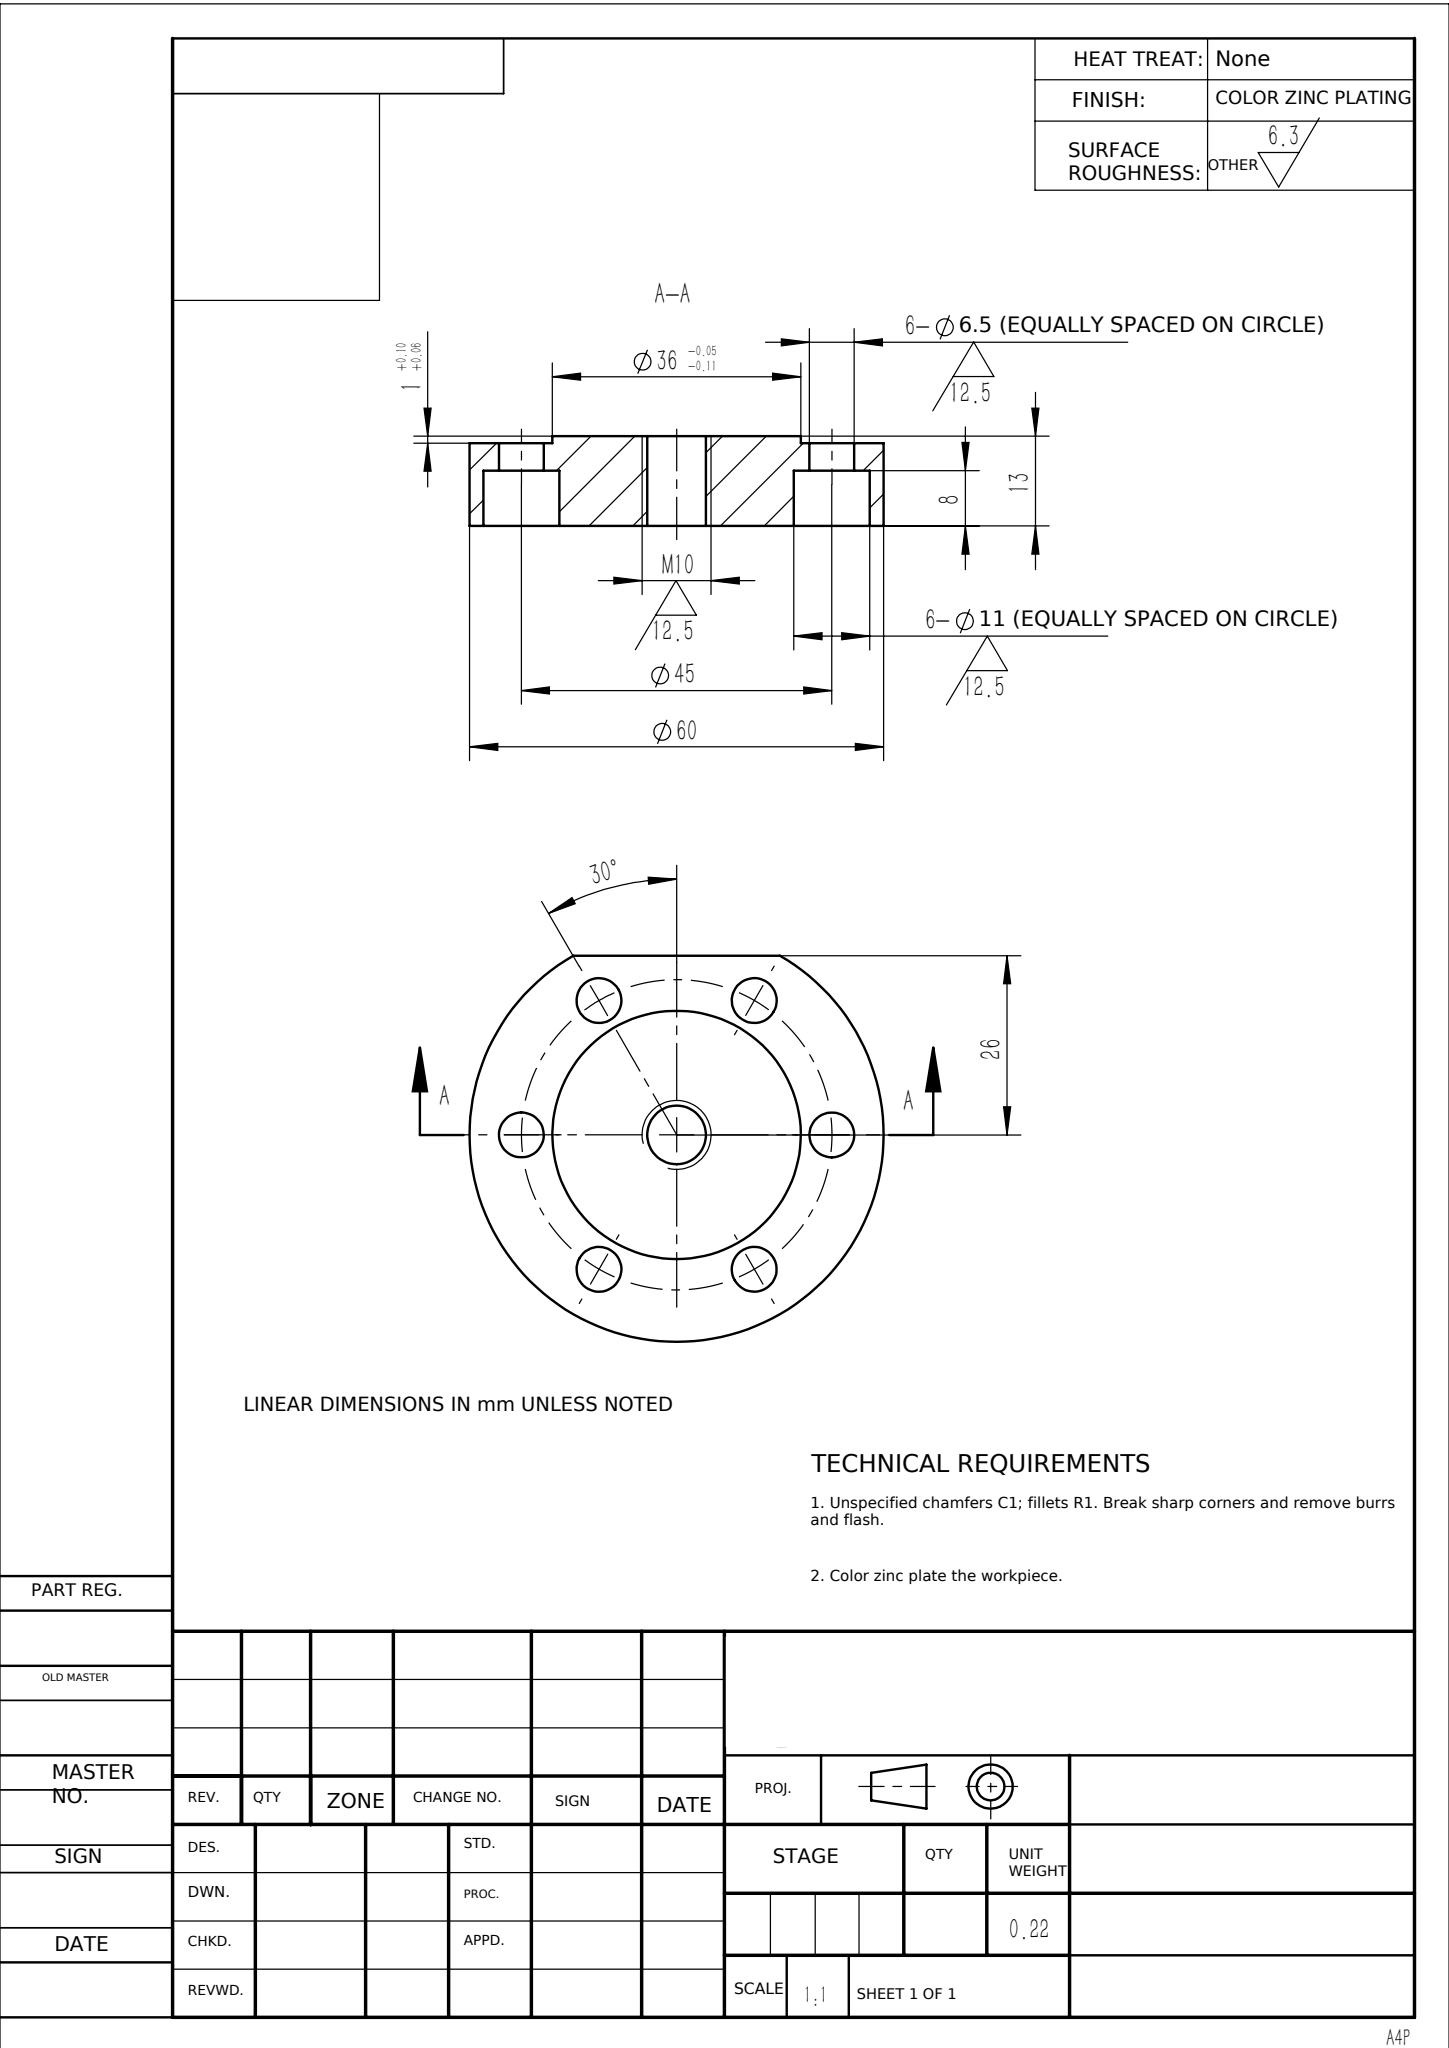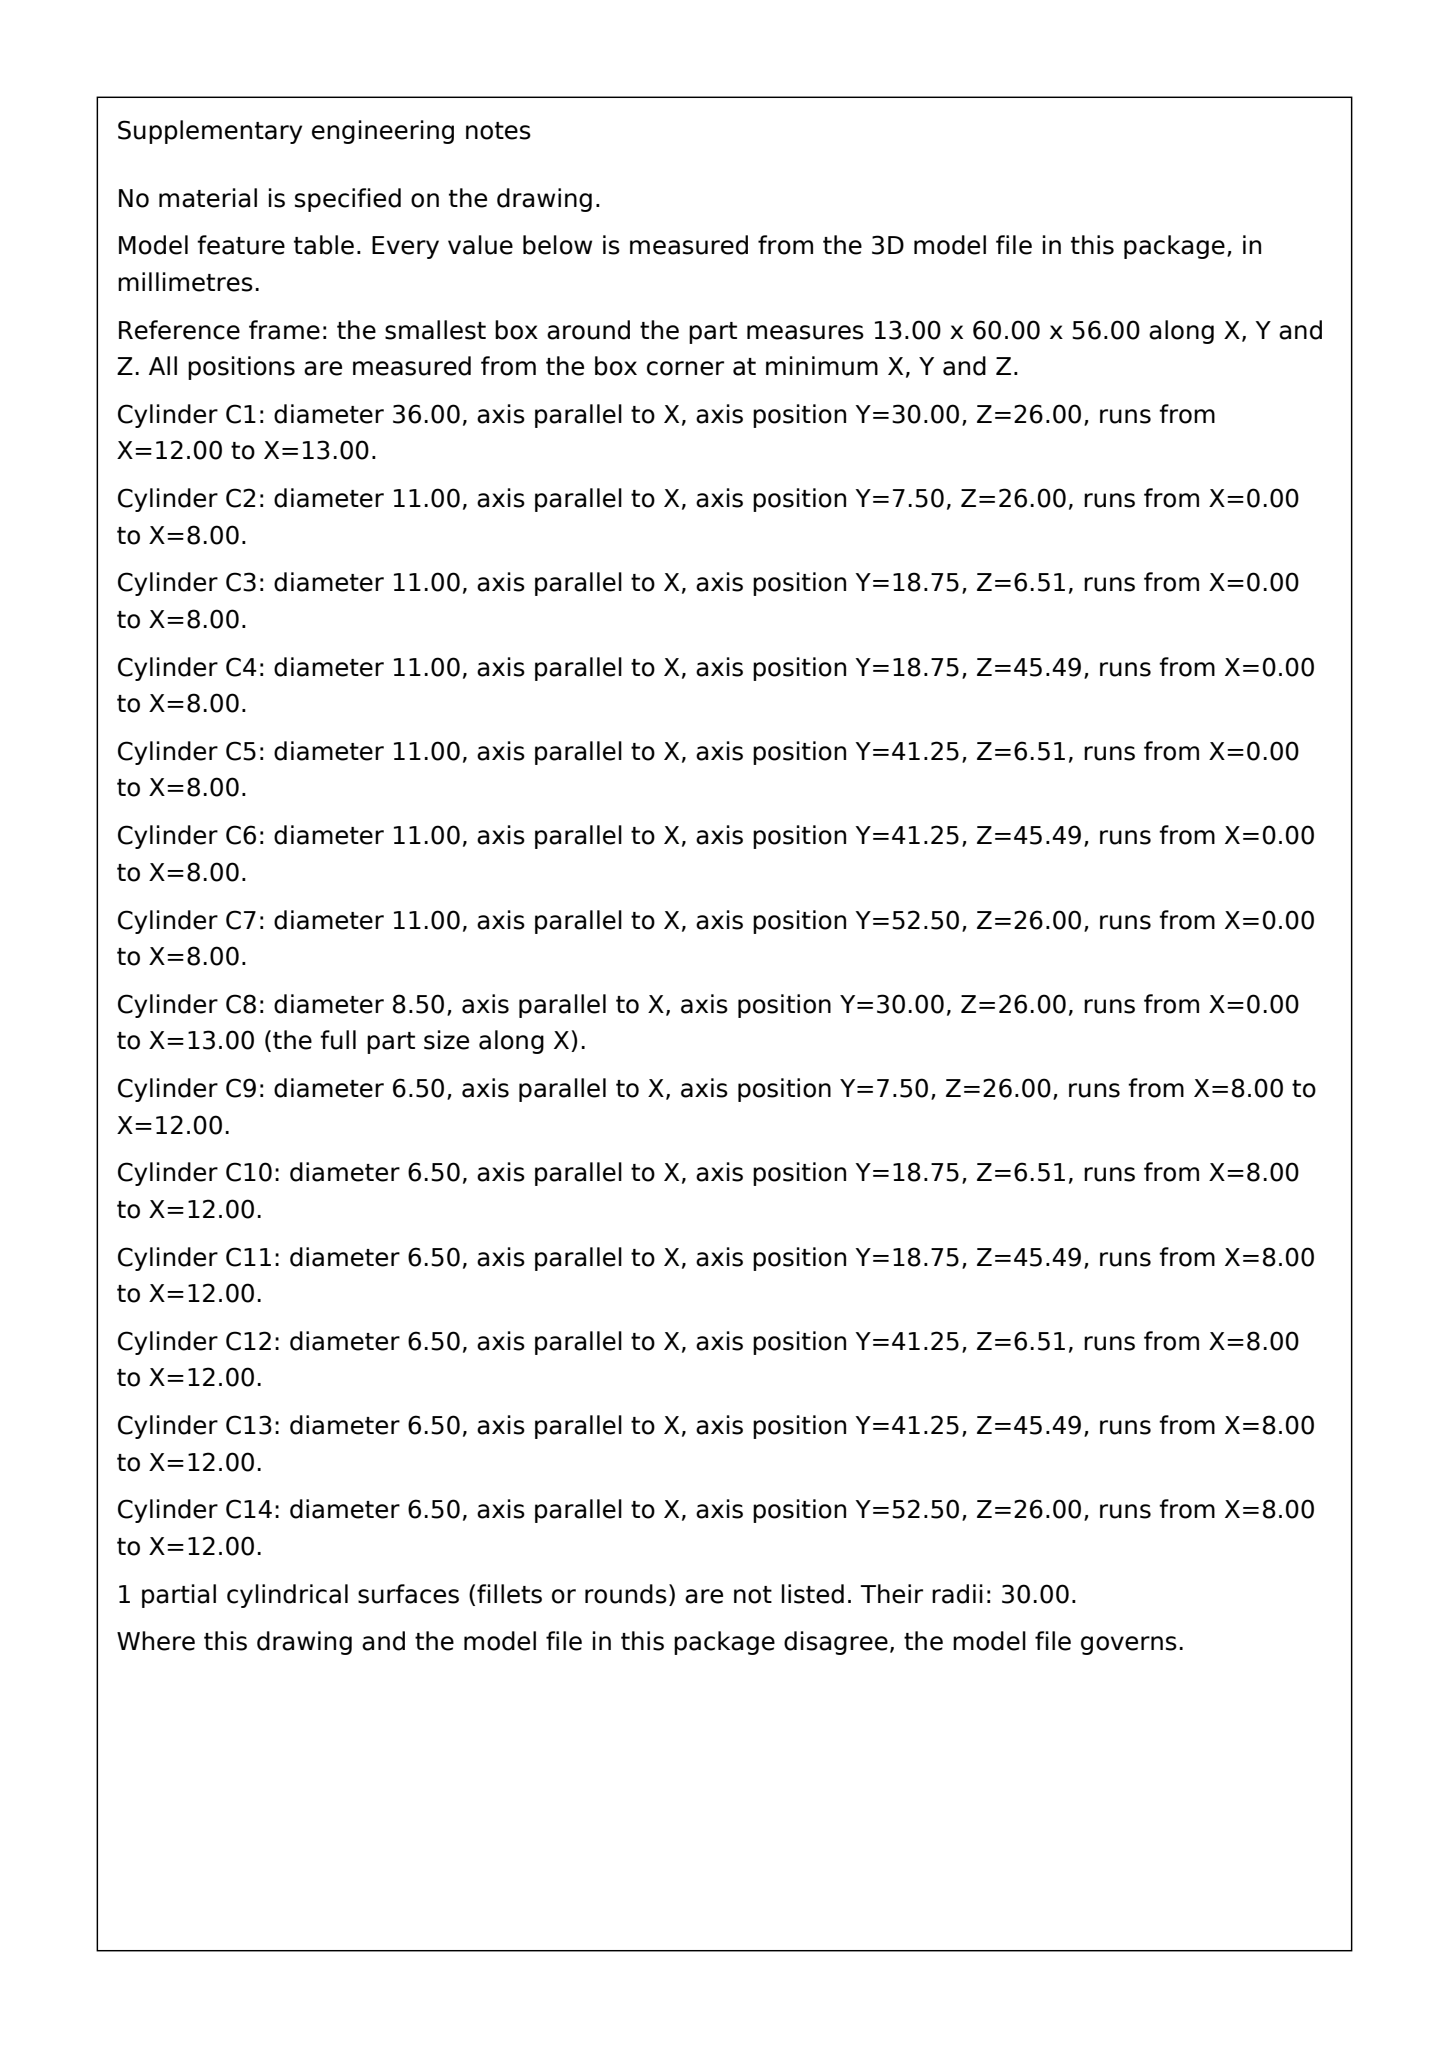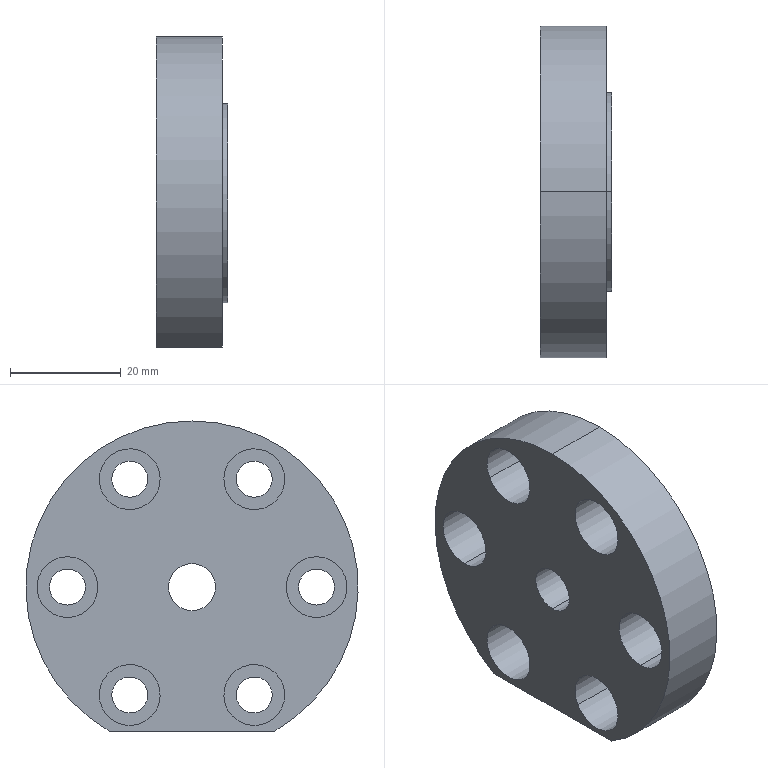Part | SolidWorks | mm | 1 solid | 40 faces | box 13 x 60 x 56 mm | volume 27880 mm3 | cylinder 30 | plane 10 | commonest cylinder face diameters 11 x12 6.5 x12 8.5 x2 60 x2 36 x2
build123d program:
from build123d import *

# Parameters (mm, degrees)
SKETCH2_R          = 3.25
CUT_EXTRUDE1_DEPTH = 45.091
CUT_EXTRUDE2_DEPTH = 45.373
M10_TAPPED_HOLE1_D = 8.5
SKETCH6_R          = 5.5
CUT_EXTRUDE3_DEPTH = 8
CIRPATTERN1_COUNT  = 6


with BuildPart() as part:
    # Sketch1 → Revolve1 (revolve)
    with BuildSketch(Plane.XY, mode=Mode.PRIVATE) as revolve1_sk:
        Polygon((0, 0), (13, 0), (13, 18), (12, 18), (12, 30), (0, 30), align=None)
    revolve(revolve1_sk.sketch.rotate(Axis((0, 0, 0), (1, 0, 0)), 90), axis=Axis((0, 0, 0), (1, 0, 0)))

    # Sketch2 → Cut-Extrude1 (cut, through all)
    with BuildSketch(Plane(origin=(12, 0, 0), x_dir=(0, 0, -1), z_dir=(1, 0, 0))):
        with Locations((0, 22.5)):
            Circle(SKETCH2_R)
    cut_extrude1 = extrude(amount=-CUT_EXTRUDE1_DEPTH, mode=Mode.SUBTRACT)

    # Sketch3 → Cut-Extrude2 (cut, through all)
    with BuildSketch(Plane.ZY):
        with BuildLine():
            Line((-26, 14.967), (-26, -14.967))
            ThreePointArc((-26, -14.967), (-30, 0), (-26, 14.967))
        make_face()
    extrude(amount=-CUT_EXTRUDE2_DEPTH, mode=Mode.SUBTRACT)

    # M10 Tapped Hole1 (through all)
    with Locations(Plane.ZY):
        with Locations((0, 0)):
            Hole(M10_TAPPED_HOLE1_D / 2)

    # Sketch6 → Cut-Extrude3 (cut)
    with BuildSketch(Plane.ZY):
        with Locations((0, 22.5)):
            Circle(SKETCH6_R)
    cut_extrude3 = extrude(amount=-CUT_EXTRUDE3_DEPTH, mode=Mode.SUBTRACT)

    # CirPattern1: Cut-Extrude1, Cut-Extrude3 ×6 about axis
    cirpattern1_axis = Axis((0, 0, 0), (1, 0, 0))
    add([cut_extrude1.rotate(cirpattern1_axis, i * 360 / CIRPATTERN1_COUNT) for i in range(1, CIRPATTERN1_COUNT)], mode=Mode.SUBTRACT)
    add([cut_extrude3.rotate(cirpattern1_axis, i * 360 / CIRPATTERN1_COUNT) for i in range(1, CIRPATTERN1_COUNT)], mode=Mode.SUBTRACT)


solid = part.part